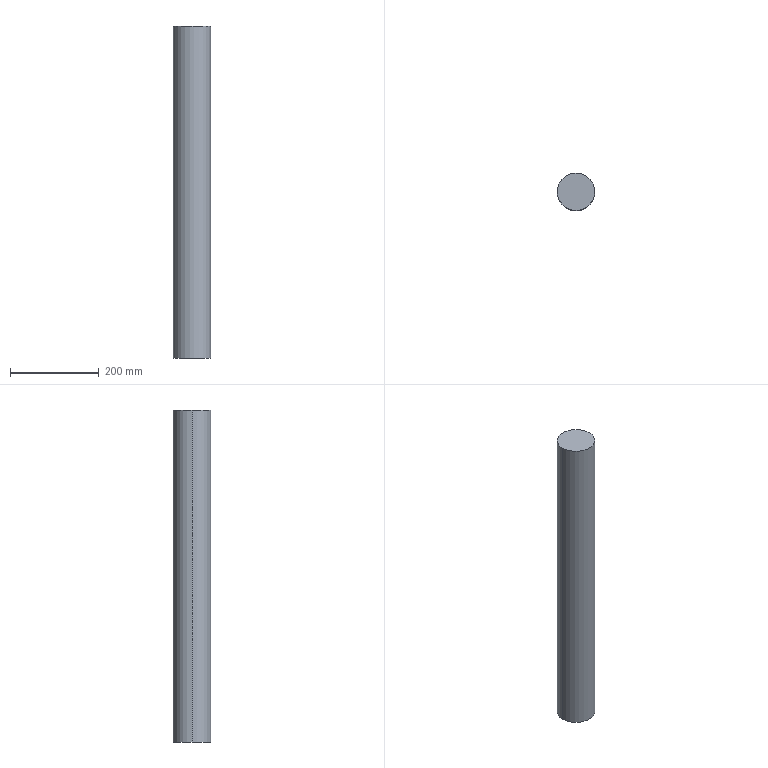Component | SolidWorks | CylinderRod1-1 | 1 solid | 4 faces | box 85 x 85 x 750 mm | volume 4255876 mm3 | cylinder 2 | plane 2 | commonest cylinder face diameters 85 x2 | material 201 Annealed Stainless Steel (SS)
build123d program:
from build123d import *

# Parameters (mm, degrees)
SKETCH1_R           = 42.5
BOSS_EXTRUDE1_DEPTH = 750


with BuildPart() as part:
    # Sketch1 → Boss-Extrude1 (new body)
    with BuildSketch(Plane.XY):
        Circle(SKETCH1_R)
    extrude(amount=BOSS_EXTRUDE1_DEPTH)


solid = part.part

# Placed as in the assembly
solid = solid.moved(Location((-7.456, 2.584, -375), (0, 0, 0)))
STEP:
#1=CARTESIAN_POINT('',(1.38,0.1017,14.764));
#2=VERTEX_POINT('',#1);
#3=CARTESIAN_POINT('',(-1.967,0.1017,14.764));
#4=VERTEX_POINT('',#3);
#5=CARTESIAN_POINT('',(-0.2935,0.1017,14.764));
#6=DIRECTION('',(0.,0.,1.));
#7=DIRECTION('',(1.,0.,0.));
#8=AXIS2_PLACEMENT_3D('',#5,#6,#7);
#9=CIRCLE('',#8,1.673);
#10=EDGE_CURVE('',#2,#4,#9,.T.);
#11=ORIENTED_EDGE('',*,*,#10,.F.);
#12=CARTESIAN_POINT('',(1.38,0.1017,-14.764));
#13=VERTEX_POINT('',#12);
#14=CARTESIAN_POINT('',(1.38,0.1017,14.764));
#15=DIRECTION('',(0.,0.,-1.));
#16=VECTOR('',#15,39.37);
#17=LINE('',#14,#16);
#18=EDGE_CURVE('',#2,#13,#17,.T.);
#19=ORIENTED_EDGE('',*,*,#18,.T.);
#20=CARTESIAN_POINT('',(-1.967,0.1017,-14.764));
#21=VERTEX_POINT('',#20);
#22=CARTESIAN_POINT('',(-0.2935,0.1017,-14.764));
#23=DIRECTION('',(0.,0.,1.));
#24=DIRECTION('',(1.,0.,0.));
#25=AXIS2_PLACEMENT_3D('',#22,#23,#24);
#26=CIRCLE('',#25,1.673);
#27=EDGE_CURVE('',#13,#21,#26,.T.);
#28=ORIENTED_EDGE('',*,*,#27,.T.);
#29=CARTESIAN_POINT('',(-1.967,0.1017,14.764));
#30=DIRECTION('',(0.,0.,-1.));
#31=VECTOR('',#30,39.37);
#32=LINE('',#29,#31);
#33=EDGE_CURVE('',#4,#21,#32,.T.);
#34=ORIENTED_EDGE('',*,*,#33,.F.);
#35=EDGE_LOOP('',(#11,#19,#28,#34));
#36=FACE_OUTER_BOUND('',#35,.T.);
#37=CARTESIAN_POINT('',(-0.2935,0.1017,14.764));
#38=DIRECTION('',(0.,0.,-1.));
#39=DIRECTION('',(-1.,0.,0.));
#40=AXIS2_PLACEMENT_3D('',#37,#38,#39);
#41=CYLINDRICAL_SURFACE('',#40,1.673);
#42=ADVANCED_FACE('',(#36),#41,.T.);
#43=ORIENTED_EDGE('',*,*,#18,.F.);
#44=CARTESIAN_POINT('',(-0.2935,0.1017,14.764));
#45=DIRECTION('',(0.,0.,1.));
#46=DIRECTION('',(1.,0.,0.));
#47=AXIS2_PLACEMENT_3D('',#44,#45,#46);
#48=CIRCLE('',#47,1.673);
#49=EDGE_CURVE('',#4,#2,#48,.T.);
#50=ORIENTED_EDGE('',*,*,#49,.F.);
#51=ORIENTED_EDGE('',*,*,#33,.T.);
#52=CARTESIAN_POINT('',(-0.2935,0.1017,-14.764));
#53=DIRECTION('',(0.,0.,1.));
#54=DIRECTION('',(1.,0.,0.));
#55=AXIS2_PLACEMENT_3D('',#52,#53,#54);
#56=CIRCLE('',#55,1.673);
#57=EDGE_CURVE('',#21,#13,#56,.T.);
#58=ORIENTED_EDGE('',*,*,#57,.T.);
#59=EDGE_LOOP('',(#43,#50,#51,#58));
#60=FACE_OUTER_BOUND('',#59,.T.);
#61=CARTESIAN_POINT('',(-0.2935,0.1017,14.764));
#62=DIRECTION('',(0.,0.,-1.));
#63=DIRECTION('',(-1.,0.,0.));
#64=AXIS2_PLACEMENT_3D('',#61,#62,#63);
#65=CYLINDRICAL_SURFACE('',#64,1.673);
#66=ADVANCED_FACE('',(#60),#65,.T.);
#67=ORIENTED_EDGE('',*,*,#49,.T.);
#68=ORIENTED_EDGE('',*,*,#10,.T.);
#69=EDGE_LOOP('',(#67,#68));
#70=FACE_OUTER_BOUND('',#69,.T.);
#71=CARTESIAN_POINT('',(-0.2935,0.1017,14.764));
#72=DIRECTION('',(0.,0.,1.));
#73=DIRECTION('',(1.,0.,0.));
#74=AXIS2_PLACEMENT_3D('',#71,#72,#73);
#75=PLANE('',#74);
#76=ADVANCED_FACE('',(#70),#75,.T.);
#77=ORIENTED_EDGE('',*,*,#57,.F.);
#78=ORIENTED_EDGE('',*,*,#27,.F.);
#79=EDGE_LOOP('',(#77,#78));
#80=FACE_OUTER_BOUND('',#79,.T.);
#81=CARTESIAN_POINT('',(-0.2935,0.1017,-14.764));
#82=DIRECTION('',(0.,0.,1.));
#83=DIRECTION('',(1.,0.,0.));
#84=AXIS2_PLACEMENT_3D('',#81,#82,#83);
#85=PLANE('',#84);
#86=ADVANCED_FACE('',(#80),#85,.F.);
#87=CLOSED_SHELL('',(#42,#66,#76,#86));
#88=MANIFOLD_SOLID_BREP('',#87);
#89=CARTESIAN_POINT('',(0.,0.,0.));
#90=DIRECTION('',(0.,0.,1.));
#91=DIRECTION('',(1.,0.,0.));
#92=AXIS2_PLACEMENT_3D('',#89,#90,#91);
#93=(LENGTH_UNIT()NAMED_UNIT(*)SI_UNIT($,.METRE.));
#94=LENGTH_MEASURE_WITH_UNIT(LENGTH_MEASURE(0.0254),#93);
#95=DIMENSIONAL_EXPONENTS(1.,0.,0.,0.,0.,0.,0.);
#96=(CONVERSION_BASED_UNIT('',#94)LENGTH_UNIT()NAMED_UNIT(#95));
#97=UNCERTAINTY_MEASURE_WITH_UNIT(LENGTH_MEASURE(0.00001),#96,'','');
#98=(NAMED_UNIT(*)PLANE_ANGLE_UNIT()SI_UNIT($,.RADIAN.));
#99=(NAMED_UNIT(*)SI_UNIT($,.STERADIAN.)SOLID_ANGLE_UNIT());
#100=(GEOMETRIC_REPRESENTATION_CONTEXT(3)GLOBAL_UNCERTAINTY_ASSIGNED_CONTEXT((#97))GLOBAL_UNIT_ASSIGNED_CONTEXT((#96,#98,#99))REPRESENTATION_CONTEXT('',''));
#101=ADVANCED_BREP_SHAPE_REPRESENTATION('',(#88,#92),#100);
#102=COLOUR_RGB('',0.7922,0.8196,0.9333);
#103=FILL_AREA_STYLE_COLOUR('',#102);
#104=FILL_AREA_STYLE('',(#103));
#105=SURFACE_STYLE_FILL_AREA(#104);
#106=SURFACE_SIDE_STYLE('',(#105));
#107=SURFACE_STYLE_USAGE(.BOTH.,#106);
#108=PRESENTATION_STYLE_ASSIGNMENT((#107));
#109=STYLED_ITEM('',(#108),#88);
#110=(LENGTH_UNIT()NAMED_UNIT(*)SI_UNIT($,.METRE.));
#111=LENGTH_MEASURE_WITH_UNIT(LENGTH_MEASURE(0.0254),#110);
#112=DIMENSIONAL_EXPONENTS(1.,0.,0.,0.,0.,0.,0.);
#113=(CONVERSION_BASED_UNIT('',#111)LENGTH_UNIT()NAMED_UNIT(#112));
#114=UNCERTAINTY_MEASURE_WITH_UNIT(LENGTH_MEASURE(0.00001),#113,'','');
#115=(NAMED_UNIT(*)PLANE_ANGLE_UNIT()SI_UNIT($,.RADIAN.));
#116=(NAMED_UNIT(*)SI_UNIT($,.STERADIAN.)SOLID_ANGLE_UNIT());
#117=(GEOMETRIC_REPRESENTATION_CONTEXT(3)GLOBAL_UNCERTAINTY_ASSIGNED_CONTEXT((#114))GLOBAL_UNIT_ASSIGNED_CONTEXT((#113,#115,#116))REPRESENTATION_CONTEXT('',''));
#118=MECHANICAL_DESIGN_GEOMETRIC_PRESENTATION_REPRESENTATION('',(#109),#117);
#119=PRESENTATION_LAYER_ASSIGNMENT('','',(#109));